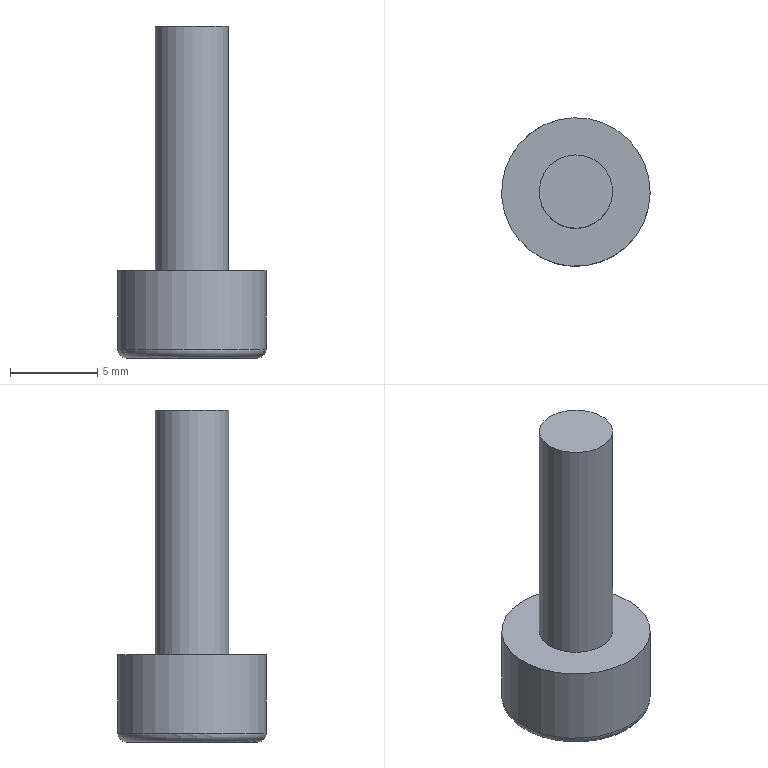Component | NX | 13_T70_1_M5X14_CAP_SCREW_5 | 1 solid | 25 faces | volume 428 mm3 | plane 15 | cone 7 | cylinder 2 | torus 1 | commonest cylinder face diameters 8.5 x1 4.2 x1